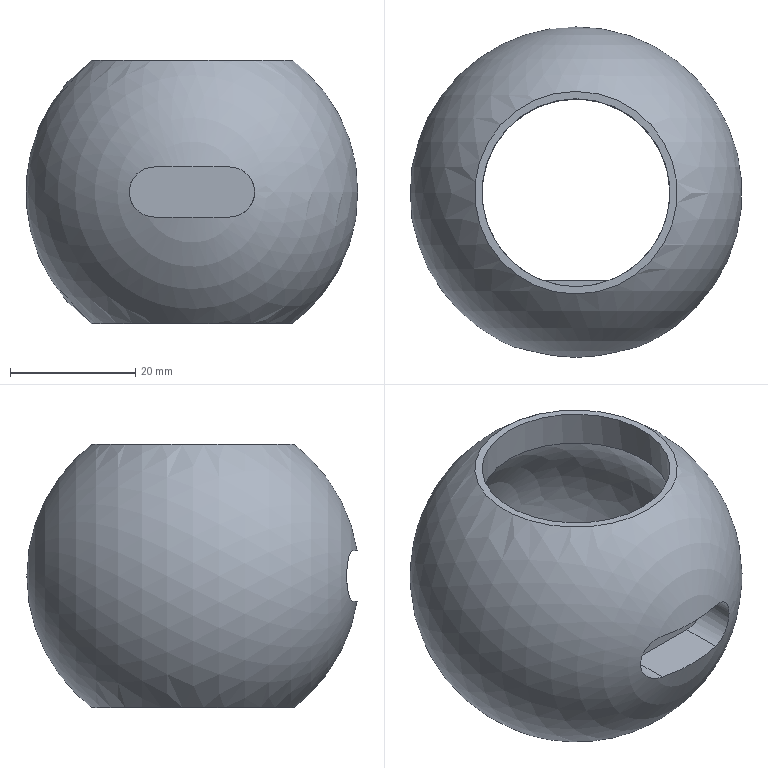Component | NX | VALVE_CORE | 1 solid | 26 faces | volume 29870 mm3 | cylinder 8 | plane 8 | spline 6 | sphere 2 | torus 2 | commonest cylinder face diameters 18 x4 30 x2 8 x2